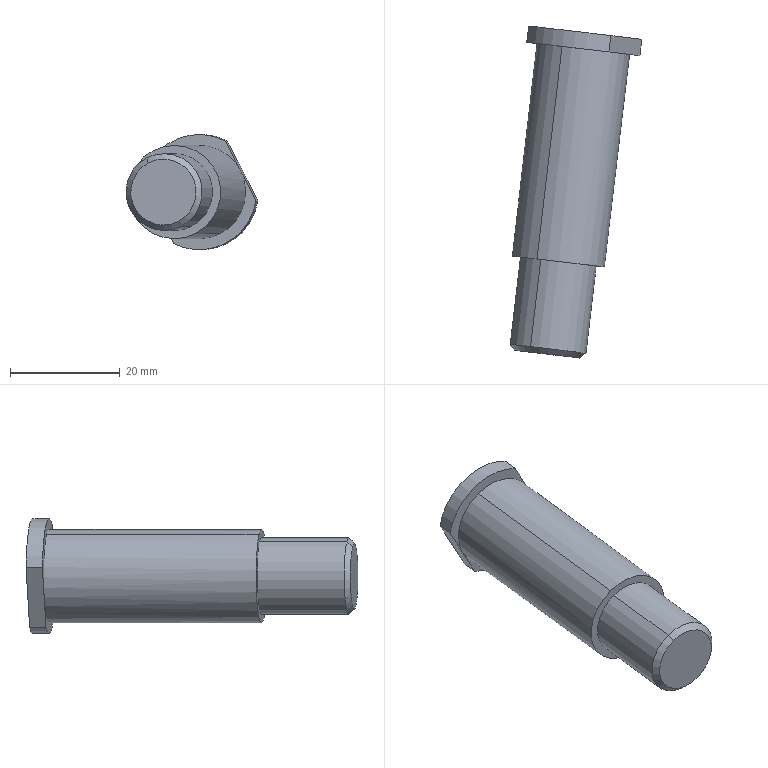Component | SolidWorks | 8TC-A17001-91-00UpperAndLowerPressAssembly-1_8TC-A17001-91-04PressureRollerAxis-1 | 1 solid | 16 faces | box 24.03 x 60.51 x 21 mm | volume 12387 mm3 | cylinder 7 | plane 7 | cone 2 | commonest cylinder face diameters 21 x3 14 x2 17 x2 | material Cr12MoV
build123d program:
from build123d import *

# Parameters (mm, degrees)
SKETCH1_R               = 10.5
BOSS_EXTRUDE1_DEPTH     = 3
SKETCH2_R               = 8.5
BOSS_EXTRUDE2_DEPTH     = 56
CUT_EXTRUDE1_DEPTH      = 61.84
CUT_EXTRUDE1_DEPTH_BACK = 61.84
SKETCH3_W               = 5
SKETCH3_H               = 5
SKETCH4_W               = 5
SKETCH4_H               = 17
CHAMFER1_SIZE           = 1


with BuildPart() as part:
    # Sketch1 → Boss-Extrude1 (new body)
    with BuildSketch(Plane(origin=(0, 0, 0), x_dir=(1, 0, 0), z_dir=(0, 1, 0))):
        with Locations(Location((0, 0, 0), (0, 0, 270))):
            Circle(SKETCH1_R)
    extrude(amount=BOSS_EXTRUDE1_DEPTH)

    # Sketch2 → Boss-Extrude2 (add)
    with BuildSketch(Plane(origin=(0, 3, 0), x_dir=(1, 0, 0), z_dir=(0, 1, 0))):
        with Locations(Location((0, 0, 0), (0, 0, 270))):
            Circle(SKETCH2_R)
    extrude(amount=BOSS_EXTRUDE2_DEPTH)

    # Sketch3 → Cut-Extrude1 (cut, two sides: drawn at the far end of the back side and taken through both)
    with BuildSketch(Plane.XY.offset(-CUT_EXTRUDE1_DEPTH_BACK)):
        with Locations((-11, 2.5)):
            Rectangle(SKETCH3_W, SKETCH3_H)
        with Locations((11, 2.5)):
            Rectangle(SKETCH3_W, SKETCH3_H)
    extrude(amount=CUT_EXTRUDE1_DEPTH + CUT_EXTRUDE1_DEPTH_BACK, mode=Mode.SUBTRACT)

    # Sketch4 → Cut-Revolve1 (revolve, cut)
    with BuildSketch(Plane.XY, mode=Mode.PRIVATE) as cut_revolve1_sk:
        with Locations((9.5, 50.5)):
            Rectangle(SKETCH4_W, SKETCH4_H)
    revolve(cut_revolve1_sk.sketch.rotate(Axis((0, 0, 0), (0, 1, 0)), 90), axis=Axis((0, 0, 0), (0, 1, 0)), mode=Mode.SUBTRACT)

    # Chamfer1
    chamfer1_edges = [part.edges().sort_by_distance(p)[0] for p in [
        (0, 59, 7),
    ]]
    chamfer(chamfer1_edges, length=CHAMFER1_SIZE)


solid = part.part

# Placed as in the assembly
solid = solid.moved(Location((3.937, -58.742, -52), (176.545, 27.162, 7.535)))
STEP:
#1=COLOUR_RGB('',0.7922,0.8196,0.9333);
#2=FILL_AREA_STYLE_COLOUR('',#1);
#3=FILL_AREA_STYLE('',(#2));
#4=SURFACE_STYLE_FILL_AREA(#3);
#5=SURFACE_SIDE_STYLE('',(#4));
#6=SURFACE_STYLE_USAGE(.BOTH.,#5);
#7=PRESENTATION_STYLE_ASSIGNMENT((#6));
#8=CARTESIAN_POINT('',(-0.2238,-4.607,-1.837));
#9=VERTEX_POINT('',#8);
#10=CARTESIAN_POINT('',(-0.008168,-4.632,-2.257));
#11=VERTEX_POINT('',#10);
#12=CARTESIAN_POINT('',(-0.116,-4.62,-2.047));
#13=DIRECTION('',(-0.1167,-0.9932,0.));
#14=DIRECTION('',(-0.4565,0.05363,0.8881));
#15=AXIS2_PLACEMENT_3D('',#12,#13,#14);
#16=CIRCLE('',#15,0.2362);
#17=EDGE_CURVE('',#9,#11,#16,.T.);
#18=ORIENTED_EDGE('',*,*,#17,.F.);
#19=CARTESIAN_POINT('',(-0.2372,-4.566,-1.802));
#20=VERTEX_POINT('',#19);
#21=CARTESIAN_POINT('',(-0.2372,-4.566,-1.802));
#22=DIRECTION('',(-0.2403,0.7402,0.628));
#23=VECTOR('',#22,39.37);
#24=LINE('',#21,#23);
#25=EDGE_CURVE('',#9,#20,#24,.T.);
#26=ORIENTED_EDGE('',*,*,#25,.T.);
#27=CARTESIAN_POINT('',(0.0144,-4.595,-2.292));
#28=VERTEX_POINT('',#27);
#29=CARTESIAN_POINT('',(-0.1114,-4.581,-2.047));
#30=DIRECTION('',(0.1167,0.9932,-0.));
#31=DIRECTION('',(-0.4565,0.05363,0.8881));
#32=AXIS2_PLACEMENT_3D('',#29,#30,#31);
#33=CIRCLE('',#32,0.2756);
#34=EDGE_CURVE('',#28,#20,#33,.T.);
#35=ORIENTED_EDGE('',*,*,#34,.F.);
#36=CARTESIAN_POINT('',(0.0144,-4.595,-2.292));
#37=DIRECTION('',(0.4053,0.6644,-0.628));
#38=VECTOR('',#37,39.37);
#39=LINE('',#36,#38);
#40=EDGE_CURVE('',#11,#28,#39,.T.);
#41=ORIENTED_EDGE('',*,*,#40,.F.);
#42=EDGE_LOOP('',(#18,#26,#35,#41));
#43=FACE_OUTER_BOUND('',#42,.T.);
#44=CARTESIAN_POINT('',(-0.1114,-4.581,-2.047));
#45=DIRECTION('',(0.1167,0.9932,-0.));
#46=DIRECTION('',(0.4565,-0.05363,-0.8881));
#47=AXIS2_PLACEMENT_3D('',#44,#45,#46);
#48=CONICAL_SURFACE('',#47,0.2756,0.7854);
#49=ADVANCED_FACE('',(#43),#48,.T.);
#50=ORIENTED_EDGE('',*,*,#34,.T.);
#51=CARTESIAN_POINT('',(-0.1637,-3.94,-1.802));
#52=VERTEX_POINT('',#51);
#53=CARTESIAN_POINT('',(0.02918,-2.298,-1.802));
#54=DIRECTION('',(0.1167,0.9932,-0.));
#55=VECTOR('',#54,39.37);
#56=LINE('',#53,#55);
#57=EDGE_CURVE('',#20,#52,#56,.T.);
#58=ORIENTED_EDGE('',*,*,#57,.T.);
#59=CARTESIAN_POINT('',(0.08789,-3.97,-2.292));
#60=VERTEX_POINT('',#59);
#61=CARTESIAN_POINT('',(-0.03792,-3.955,-2.047));
#62=DIRECTION('',(0.1167,0.9932,-0.));
#63=DIRECTION('',(0.4565,-0.05363,-0.8881));
#64=AXIS2_PLACEMENT_3D('',#61,#62,#63);
#65=CIRCLE('',#64,0.2756);
#66=EDGE_CURVE('',#60,#52,#65,.T.);
#67=ORIENTED_EDGE('',*,*,#66,.F.);
#68=CARTESIAN_POINT('',(0.2808,-2.327,-2.292));
#69=DIRECTION('',(0.1167,0.9932,-0.));
#70=VECTOR('',#69,39.37);
#71=LINE('',#68,#70);
#72=EDGE_CURVE('',#28,#60,#71,.T.);
#73=ORIENTED_EDGE('',*,*,#72,.F.);
#74=EDGE_LOOP('',(#50,#58,#67,#73));
#75=FACE_OUTER_BOUND('',#74,.T.);
#76=CARTESIAN_POINT('',(0.155,-2.313,-2.047));
#77=DIRECTION('',(0.1167,0.9932,-0.));
#78=DIRECTION('',(0.4565,-0.05363,-0.8881));
#79=AXIS2_PLACEMENT_3D('',#76,#77,#78);
#80=CYLINDRICAL_SURFACE('',#79,0.2756);
#81=ADVANCED_FACE('',(#75),#80,.T.);
#82=CARTESIAN_POINT('',(0.1148,-3.973,-2.344));
#83=VERTEX_POINT('',#82);
#84=CARTESIAN_POINT('',(-0.1907,-3.937,-1.75));
#85=VERTEX_POINT('',#84);
#86=CARTESIAN_POINT('',(-0.03792,-3.955,-2.047));
#87=DIRECTION('',(0.1167,0.9932,-0.));
#88=DIRECTION('',(0.4565,-0.05363,-0.8881));
#89=AXIS2_PLACEMENT_3D('',#86,#87,#88);
#90=CIRCLE('',#89,0.3346);
#91=EDGE_CURVE('',#83,#85,#90,.T.);
#92=ORIENTED_EDGE('',*,*,#91,.T.);
#93=CARTESIAN_POINT('',(-0.01156,-2.412,-1.75));
#94=VERTEX_POINT('',#93);
#95=CARTESIAN_POINT('',(-0.2688,-4.602,-1.75));
#96=DIRECTION('',(0.1167,0.9932,-0.));
#97=VECTOR('',#96,39.37);
#98=LINE('',#95,#97);
#99=EDGE_CURVE('',#85,#94,#98,.T.);
#100=ORIENTED_EDGE('',*,*,#99,.T.);
#101=CARTESIAN_POINT('',(-0.154,-2.395,-2.201));
#102=VERTEX_POINT('',#101);
#103=CARTESIAN_POINT('',(0.1412,-2.43,-2.047));
#104=DIRECTION('',(-0.1167,-0.9932,0.));
#105=DIRECTION('',(-0.4565,0.05363,0.8881));
#106=AXIS2_PLACEMENT_3D('',#103,#104,#105);
#107=CIRCLE('',#106,0.3346);
#108=EDGE_CURVE('',#94,#102,#107,.T.);
#109=ORIENTED_EDGE('',*,*,#108,.T.);
#110=CARTESIAN_POINT('',(0.294,-2.448,-2.344));
#111=VERTEX_POINT('',#110);
#112=CARTESIAN_POINT('',(0.1412,-2.43,-2.047));
#113=DIRECTION('',(-0.1167,-0.9932,0.));
#114=DIRECTION('',(-0.4565,0.05363,0.8881));
#115=AXIS2_PLACEMENT_3D('',#112,#113,#114);
#116=CIRCLE('',#115,0.3346);
#117=EDGE_CURVE('',#102,#111,#116,.T.);
#118=ORIENTED_EDGE('',*,*,#117,.T.);
#119=CARTESIAN_POINT('',(0.03676,-4.638,-2.344));
#120=DIRECTION('',(0.1167,0.9932,-0.));
#121=VECTOR('',#120,39.37);
#122=LINE('',#119,#121);
#123=EDGE_CURVE('',#83,#111,#122,.T.);
#124=ORIENTED_EDGE('',*,*,#123,.F.);
#125=EDGE_LOOP('',(#92,#100,#109,#118,#124));
#126=FACE_OUTER_BOUND('',#125,.T.);
#127=CARTESIAN_POINT('',(-0.116,-4.62,-2.047));
#128=DIRECTION('',(0.1167,0.9932,-0.));
#129=DIRECTION('',(0.4565,-0.05363,-0.8881));
#130=AXIS2_PLACEMENT_3D('',#127,#128,#129);
#131=CYLINDRICAL_SURFACE('',#130,0.3346);
#132=ADVANCED_FACE('',(#126),#131,.T.);
#133=CARTESIAN_POINT('',(0.3299,-2.452,-2.414));
#134=VERTEX_POINT('',#133);
#135=CARTESIAN_POINT('',(0.5472,-2.478,-2.109));
#136=VERTEX_POINT('',#135);
#137=CARTESIAN_POINT('',(0.1412,-2.43,-2.047));
#138=DIRECTION('',(-0.1167,-0.9932,0.));
#139=DIRECTION('',(-0.4565,0.05363,0.8881));
#140=AXIS2_PLACEMENT_3D('',#137,#138,#139);
#141=CIRCLE('',#140,0.4134);
#142=EDGE_CURVE('',#134,#136,#141,.T.);
#143=ORIENTED_EDGE('',*,*,#142,.F.);
#144=CARTESIAN_POINT('',(0.3437,-2.335,-2.414));
#145=VERTEX_POINT('',#144);
#146=CARTESIAN_POINT('',(0.3299,-2.452,-2.414));
#147=DIRECTION('',(0.1167,0.9932,-0.));
#148=VECTOR('',#147,39.37);
#149=LINE('',#146,#148);
#150=EDGE_CURVE('',#134,#145,#149,.T.);
#151=ORIENTED_EDGE('',*,*,#150,.T.);
#152=CARTESIAN_POINT('',(0.561,-2.36,-2.109));
#153=VERTEX_POINT('',#152);
#154=CARTESIAN_POINT('',(0.155,-2.313,-2.047));
#155=DIRECTION('',(-0.1167,-0.9932,0.));
#156=DIRECTION('',(-0.4565,0.05363,0.8881));
#157=AXIS2_PLACEMENT_3D('',#154,#155,#156);
#158=CIRCLE('',#157,0.4134);
#159=EDGE_CURVE('',#145,#153,#158,.T.);
#160=ORIENTED_EDGE('',*,*,#159,.T.);
#161=CARTESIAN_POINT('',(0.5472,-2.478,-2.109));
#162=DIRECTION('',(-0.1167,-0.9932,0.));
#163=VECTOR('',#162,39.37);
#164=LINE('',#161,#163);
#165=EDGE_CURVE('',#153,#136,#164,.T.);
#166=ORIENTED_EDGE('',*,*,#165,.T.);
#167=EDGE_LOOP('',(#143,#151,#160,#166));
#168=FACE_OUTER_BOUND('',#167,.T.);
#169=CARTESIAN_POINT('',(0.1412,-2.43,-2.047));
#170=DIRECTION('',(0.1167,0.9932,-0.));
#171=DIRECTION('',(0.4565,-0.05363,-0.8881));
#172=AXIS2_PLACEMENT_3D('',#169,#170,#171);
#173=CYLINDRICAL_SURFACE('',#172,0.4134);
#174=ADVANCED_FACE('',(#168),#173,.T.);
#175=ORIENTED_EDGE('',*,*,#150,.F.);
#176=CARTESIAN_POINT('',(-0.04317,-2.408,-2.417));
#177=VERTEX_POINT('',#176);
#178=CARTESIAN_POINT('',(0.1412,-2.43,-2.047));
#179=DIRECTION('',(-0.1167,-0.9932,0.));
#180=DIRECTION('',(-0.4565,0.05363,0.8881));
#181=AXIS2_PLACEMENT_3D('',#178,#179,#180);
#182=CIRCLE('',#181,0.4134);
#183=EDGE_CURVE('',#177,#134,#182,.T.);
#184=ORIENTED_EDGE('',*,*,#183,.F.);
#185=CARTESIAN_POINT('',(-0.02939,-2.291,-2.417));
#186=VERTEX_POINT('',#185);
#187=CARTESIAN_POINT('',(-0.04317,-2.408,-2.417));
#188=DIRECTION('',(0.1167,0.9932,-0.));
#189=VECTOR('',#188,39.37);
#190=LINE('',#187,#189);
#191=EDGE_CURVE('',#177,#186,#190,.T.);
#192=ORIENTED_EDGE('',*,*,#191,.T.);
#193=CARTESIAN_POINT('',(0.155,-2.313,-2.047));
#194=DIRECTION('',(-0.1167,-0.9932,0.));
#195=DIRECTION('',(-0.4565,0.05363,0.8881));
#196=AXIS2_PLACEMENT_3D('',#193,#194,#195);
#197=CIRCLE('',#196,0.4134);
#198=EDGE_CURVE('',#186,#145,#197,.T.);
#199=ORIENTED_EDGE('',*,*,#198,.T.);
#200=EDGE_LOOP('',(#175,#184,#192,#199));
#201=FACE_OUTER_BOUND('',#200,.T.);
#202=CARTESIAN_POINT('',(0.1412,-2.43,-2.047));
#203=DIRECTION('',(0.1167,0.9932,-0.));
#204=DIRECTION('',(0.4565,-0.05363,-0.8881));
#205=AXIS2_PLACEMENT_3D('',#202,#203,#204);
#206=CYLINDRICAL_SURFACE('',#205,0.4134);
#207=ADVANCED_FACE('',(#201),#206,.T.);
#208=CARTESIAN_POINT('',(-0.154,-2.395,-2.201));
#209=DIRECTION('',(-0.4565,0.05363,0.8881));
#210=VECTOR('',#209,39.37);
#211=LINE('',#208,#210);
#212=EDGE_CURVE('',#177,#102,#211,.T.);
#213=ORIENTED_EDGE('',*,*,#212,.F.);
#214=ORIENTED_EDGE('',*,*,#183,.T.);
#215=ORIENTED_EDGE('',*,*,#142,.T.);
#216=CARTESIAN_POINT('',(0.4364,-2.465,-1.893));
#217=VERTEX_POINT('',#216);
#218=CARTESIAN_POINT('',(0.4364,-2.465,-1.893));
#219=DIRECTION('',(0.4565,-0.05363,-0.8881));
#220=VECTOR('',#219,39.37);
#221=LINE('',#218,#220);
#222=EDGE_CURVE('',#217,#136,#221,.T.);
#223=ORIENTED_EDGE('',*,*,#222,.F.);
#224=CARTESIAN_POINT('',(0.1412,-2.43,-2.047));
#225=DIRECTION('',(-0.1167,-0.9932,0.));
#226=DIRECTION('',(-0.4565,0.05363,0.8881));
#227=AXIS2_PLACEMENT_3D('',#224,#225,#226);
#228=CIRCLE('',#227,0.3346);
#229=EDGE_CURVE('',#111,#217,#228,.T.);
#230=ORIENTED_EDGE('',*,*,#229,.F.);
#231=ORIENTED_EDGE('',*,*,#117,.F.);
#232=EDGE_LOOP('',(#213,#214,#215,#223,#230,#231));
#233=FACE_OUTER_BOUND('',#232,.T.);
#234=CARTESIAN_POINT('',(0.1412,-2.43,-2.047));
#235=DIRECTION('',(-0.1167,-0.9932,-0.));
#236=DIRECTION('',(-0.4565,0.05363,0.8881));
#237=AXIS2_PLACEMENT_3D('',#234,#235,#236);
#238=PLANE('',#237);
#239=ADVANCED_FACE('',(#233),#238,.T.);
#240=CARTESIAN_POINT('',(0.3394,-2.334,-1.678));
#241=VERTEX_POINT('',#240);
#242=CARTESIAN_POINT('',(-0.251,-2.265,-1.986));
#243=VERTEX_POINT('',#242);
#244=CARTESIAN_POINT('',(0.155,-2.313,-2.047));
#245=DIRECTION('',(-0.1167,-0.9932,0.));
#246=DIRECTION('',(-0.4565,0.05363,0.8881));
#247=AXIS2_PLACEMENT_3D('',#244,#245,#246);
#248=CIRCLE('',#247,0.4134);
#249=EDGE_CURVE('',#241,#243,#248,.T.);
#250=ORIENTED_EDGE('',*,*,#249,.T.);
#251=CARTESIAN_POINT('',(-0.2647,-2.382,-1.986));
#252=VERTEX_POINT('',#251);
#253=CARTESIAN_POINT('',(-0.2647,-2.382,-1.986));
#254=DIRECTION('',(-0.1167,-0.9932,0.));
#255=VECTOR('',#254,39.37);
#256=LINE('',#253,#255);
#257=EDGE_CURVE('',#243,#252,#256,.T.);
#258=ORIENTED_EDGE('',*,*,#257,.T.);
#259=CARTESIAN_POINT('',(0.3256,-2.452,-1.678));
#260=VERTEX_POINT('',#259);
#261=CARTESIAN_POINT('',(0.1412,-2.43,-2.047));
#262=DIRECTION('',(-0.1167,-0.9932,0.));
#263=DIRECTION('',(-0.4565,0.05363,0.8881));
#264=AXIS2_PLACEMENT_3D('',#261,#262,#263);
#265=CIRCLE('',#264,0.4134);
#266=EDGE_CURVE('',#260,#252,#265,.T.);
#267=ORIENTED_EDGE('',*,*,#266,.F.);
#268=CARTESIAN_POINT('',(0.3256,-2.452,-1.678));
#269=DIRECTION('',(0.1167,0.9932,-0.));
#270=VECTOR('',#269,39.37);
#271=LINE('',#268,#270);
#272=EDGE_CURVE('',#260,#241,#271,.T.);
#273=ORIENTED_EDGE('',*,*,#272,.T.);
#274=EDGE_LOOP('',(#250,#258,#267,#273));
#275=FACE_OUTER_BOUND('',#274,.T.);
#276=CARTESIAN_POINT('',(0.1412,-2.43,-2.047));
#277=DIRECTION('',(0.1167,0.9932,-0.));
#278=DIRECTION('',(0.4565,-0.05363,-0.8881));
#279=AXIS2_PLACEMENT_3D('',#276,#277,#278);
#280=CYLINDRICAL_SURFACE('',#279,0.4134);
#281=ADVANCED_FACE('',(#275),#280,.T.);
#282=CARTESIAN_POINT('',(-0.154,-2.395,-2.201));
#283=DIRECTION('',(-0.4565,0.05363,0.8881));
#284=VECTOR('',#283,39.37);
#285=LINE('',#282,#284);
#286=EDGE_CURVE('',#102,#252,#285,.T.);
#287=ORIENTED_EDGE('',*,*,#286,.F.);
#288=ORIENTED_EDGE('',*,*,#108,.F.);
#289=CARTESIAN_POINT('',(0.1412,-2.43,-2.047));
#290=DIRECTION('',(-0.1167,-0.9932,0.));
#291=DIRECTION('',(-0.4565,0.05363,0.8881));
#292=AXIS2_PLACEMENT_3D('',#289,#290,#291);
#293=CIRCLE('',#292,0.3346);
#294=EDGE_CURVE('',#217,#94,#293,.T.);
#295=ORIENTED_EDGE('',*,*,#294,.F.);
#296=CARTESIAN_POINT('',(0.4364,-2.465,-1.893));
#297=DIRECTION('',(0.4565,-0.05363,-0.8881));
#298=VECTOR('',#297,39.37);
#299=LINE('',#296,#298);
#300=EDGE_CURVE('',#260,#217,#299,.T.);
#301=ORIENTED_EDGE('',*,*,#300,.F.);
#302=ORIENTED_EDGE('',*,*,#266,.T.);
#303=EDGE_LOOP('',(#287,#288,#295,#301,#302));
#304=FACE_OUTER_BOUND('',#303,.T.);
#305=CARTESIAN_POINT('',(0.1412,-2.43,-2.047));
#306=DIRECTION('',(-0.1167,-0.9932,-0.));
#307=DIRECTION('',(-0.4565,0.05363,0.8881));
#308=AXIS2_PLACEMENT_3D('',#305,#306,#307);
#309=PLANE('',#308);
#310=ADVANCED_FACE('',(#304),#309,.T.);
#311=ORIENTED_EDGE('',*,*,#198,.F.);
#312=CARTESIAN_POINT('',(0.04854,-2.3,-2.568));
#313=DIRECTION('',(-0.4565,0.05363,0.8881));
#314=VECTOR('',#313,39.37);
#315=LINE('',#312,#314);
#316=EDGE_CURVE('',#186,#243,#315,.T.);
#317=ORIENTED_EDGE('',*,*,#316,.T.);
#318=ORIENTED_EDGE('',*,*,#249,.F.);
#319=CARTESIAN_POINT('',(0.6389,-2.37,-2.261));
#320=DIRECTION('',(-0.4565,0.05363,0.8881));
#321=VECTOR('',#320,39.37);
#322=LINE('',#319,#321);
#323=EDGE_CURVE('',#153,#241,#322,.T.);
#324=ORIENTED_EDGE('',*,*,#323,.F.);
#325=ORIENTED_EDGE('',*,*,#159,.F.);
#326=EDGE_LOOP('',(#311,#317,#318,#324,#325));
#327=FACE_OUTER_BOUND('',#326,.T.);
#328=CARTESIAN_POINT('',(0.155,-2.313,-2.047));
#329=DIRECTION('',(-0.1167,-0.9932,-0.));
#330=DIRECTION('',(-0.4565,0.05363,0.8881));
#331=AXIS2_PLACEMENT_3D('',#328,#329,#330);
#332=PLANE('',#331);
#333=ADVANCED_FACE('',(#327),#332,.F.);
#334=ORIENTED_EDGE('',*,*,#99,.F.);
#335=CARTESIAN_POINT('',(-0.03792,-3.955,-2.047));
#336=DIRECTION('',(0.1167,0.9932,-0.));
#337=DIRECTION('',(0.4565,-0.05363,-0.8881));
#338=AXIS2_PLACEMENT_3D('',#335,#336,#337);
#339=CIRCLE('',#338,0.3346);
#340=EDGE_CURVE('',#85,#83,#339,.T.);
#341=ORIENTED_EDGE('',*,*,#340,.T.);
#342=ORIENTED_EDGE('',*,*,#123,.T.);
#343=ORIENTED_EDGE('',*,*,#229,.T.);
#344=ORIENTED_EDGE('',*,*,#294,.T.);
#345=EDGE_LOOP('',(#334,#341,#342,#343,#344));
#346=FACE_OUTER_BOUND('',#345,.T.);
#347=CARTESIAN_POINT('',(-0.116,-4.62,-2.047));
#348=DIRECTION('',(0.1167,0.9932,-0.));
#349=DIRECTION('',(0.4565,-0.05363,-0.8881));
#350=AXIS2_PLACEMENT_3D('',#347,#348,#349);
#351=CYLINDRICAL_SURFACE('',#350,0.3346);
#352=ADVANCED_FACE('',(#346),#351,.T.);
#353=ORIENTED_EDGE('',*,*,#300,.T.);
#354=ORIENTED_EDGE('',*,*,#222,.T.);
#355=ORIENTED_EDGE('',*,*,#165,.F.);
#356=ORIENTED_EDGE('',*,*,#323,.T.);
#357=ORIENTED_EDGE('',*,*,#272,.F.);
#358=EDGE_LOOP('',(#353,#354,#355,#356,#357));
#359=FACE_OUTER_BOUND('',#358,.T.);
#360=CARTESIAN_POINT('',(0.6159,-2.565,-2.261));
#361=DIRECTION('',(-0.882,0.1036,-0.4596));
#362=DIRECTION('',(0.4565,-0.05363,-0.8881));
#363=AXIS2_PLACEMENT_3D('',#360,#361,#362);
#364=PLANE('',#363);
#365=ADVANCED_FACE('',(#359),#364,.F.);
#366=ORIENTED_EDGE('',*,*,#212,.T.);
#367=ORIENTED_EDGE('',*,*,#286,.T.);
#368=ORIENTED_EDGE('',*,*,#257,.F.);
#369=ORIENTED_EDGE('',*,*,#316,.F.);
#370=ORIENTED_EDGE('',*,*,#191,.F.);
#371=EDGE_LOOP('',(#366,#367,#368,#369,#370));
#372=FACE_OUTER_BOUND('',#371,.T.);
#373=CARTESIAN_POINT('',(0.02557,-2.496,-2.568));
#374=DIRECTION('',(0.882,-0.1036,0.4596));
#375=DIRECTION('',(-0.4565,0.05363,0.8881));
#376=AXIS2_PLACEMENT_3D('',#373,#374,#375);
#377=PLANE('',#376);
#378=ADVANCED_FACE('',(#372),#377,.F.);
#379=ORIENTED_EDGE('',*,*,#66,.T.);
#380=CARTESIAN_POINT('',(-0.03792,-3.955,-2.047));
#381=DIRECTION('',(0.1167,0.9932,-0.));
#382=DIRECTION('',(0.4565,-0.05363,-0.8881));
#383=AXIS2_PLACEMENT_3D('',#380,#381,#382);
#384=CIRCLE('',#383,0.2756);
#385=EDGE_CURVE('',#52,#60,#384,.T.);
#386=ORIENTED_EDGE('',*,*,#385,.T.);
#387=EDGE_LOOP('',(#379,#386));
#388=FACE_BOUND('',#387,.T.);
#389=ORIENTED_EDGE('',*,*,#91,.F.);
#390=ORIENTED_EDGE('',*,*,#340,.F.);
#391=EDGE_LOOP('',(#389,#390));
#392=FACE_OUTER_BOUND('',#391,.T.);
#393=CARTESIAN_POINT('',(-0.281,-3.926,-2.174));
#394=DIRECTION('',(0.1167,0.9932,0.));
#395=DIRECTION('',(0.4565,-0.05363,-0.8881));
#396=AXIS2_PLACEMENT_3D('',#393,#394,#395);
#397=PLANE('',#396);
#398=ADVANCED_FACE('',(#388,#392),#397,.F.);
#399=ORIENTED_EDGE('',*,*,#57,.F.);
#400=CARTESIAN_POINT('',(-0.1114,-4.581,-2.047));
#401=DIRECTION('',(0.1167,0.9932,-0.));
#402=DIRECTION('',(-0.4565,0.05363,0.8881));
#403=AXIS2_PLACEMENT_3D('',#400,#401,#402);
#404=CIRCLE('',#403,0.2756);
#405=EDGE_CURVE('',#20,#28,#404,.T.);
#406=ORIENTED_EDGE('',*,*,#405,.T.);
#407=ORIENTED_EDGE('',*,*,#72,.T.);
#408=ORIENTED_EDGE('',*,*,#385,.F.);
#409=EDGE_LOOP('',(#399,#406,#407,#408));
#410=FACE_OUTER_BOUND('',#409,.T.);
#411=CARTESIAN_POINT('',(0.155,-2.313,-2.047));
#412=DIRECTION('',(0.1167,0.9932,-0.));
#413=DIRECTION('',(0.4565,-0.05363,-0.8881));
#414=AXIS2_PLACEMENT_3D('',#411,#412,#413);
#415=CYLINDRICAL_SURFACE('',#414,0.2756);
#416=ADVANCED_FACE('',(#410),#415,.T.);
#417=CARTESIAN_POINT('',(-0.116,-4.62,-2.047));
#418=DIRECTION('',(-0.1167,-0.9932,0.));
#419=DIRECTION('',(-0.4565,0.05363,0.8881));
#420=AXIS2_PLACEMENT_3D('',#417,#418,#419);
#421=CIRCLE('',#420,0.2362);
#422=EDGE_CURVE('',#11,#9,#421,.T.);
#423=ORIENTED_EDGE('',*,*,#422,.T.);
#424=ORIENTED_EDGE('',*,*,#17,.T.);
#425=EDGE_LOOP('',(#423,#424));
#426=FACE_OUTER_BOUND('',#425,.T.);
#427=CARTESIAN_POINT('',(-0.116,-4.62,-2.047));
#428=DIRECTION('',(-0.1167,-0.9932,-0.));
#429=DIRECTION('',(-0.4565,0.05363,0.8881));
#430=AXIS2_PLACEMENT_3D('',#427,#428,#429);
#431=PLANE('',#430);
#432=ADVANCED_FACE('',(#426),#431,.T.);
#433=ORIENTED_EDGE('',*,*,#25,.F.);
#434=ORIENTED_EDGE('',*,*,#422,.F.);
#435=ORIENTED_EDGE('',*,*,#40,.T.);
#436=ORIENTED_EDGE('',*,*,#405,.F.);
#437=EDGE_LOOP('',(#433,#434,#435,#436));
#438=FACE_OUTER_BOUND('',#437,.T.);
#439=CARTESIAN_POINT('',(-0.1114,-4.581,-2.047));
#440=DIRECTION('',(0.1167,0.9932,-0.));
#441=DIRECTION('',(0.4565,-0.05363,-0.8881));
#442=AXIS2_PLACEMENT_3D('',#439,#440,#441);
#443=CONICAL_SURFACE('',#442,0.2756,0.7854);
#444=ADVANCED_FACE('',(#438),#443,.T.);
#445=CLOSED_SHELL('',(#49,#81,#132,#174,#207,#239,#281,#310,#333,#352,#365,#378,#398,#416,#432,#444));
#446=MANIFOLD_SOLID_BREP('',#445);
#447=STYLED_ITEM('',(#7),#446);
#448=(LENGTH_UNIT()NAMED_UNIT(*)SI_UNIT($,.METRE.));
#449=LENGTH_MEASURE_WITH_UNIT(LENGTH_MEASURE(0.0254),#448);
#450=DIMENSIONAL_EXPONENTS(1.,0.,0.,0.,0.,0.,0.);
#451=(CONVERSION_BASED_UNIT('',#449)LENGTH_UNIT()NAMED_UNIT(#450));
#452=UNCERTAINTY_MEASURE_WITH_UNIT(LENGTH_MEASURE(0.00001),#451,'','');
#453=(NAMED_UNIT(*)PLANE_ANGLE_UNIT()SI_UNIT($,.RADIAN.));
#454=(NAMED_UNIT(*)SI_UNIT($,.STERADIAN.)SOLID_ANGLE_UNIT());
#455=(GEOMETRIC_REPRESENTATION_CONTEXT(3)GLOBAL_UNCERTAINTY_ASSIGNED_CONTEXT((#452))GLOBAL_UNIT_ASSIGNED_CONTEXT((#451,#453,#454))REPRESENTATION_CONTEXT('',''));
#456=MECHANICAL_DESIGN_GEOMETRIC_PRESENTATION_REPRESENTATION('',(#447),#455);
#457=CARTESIAN_POINT('',(0.,0.,0.));
#458=DIRECTION('',(0.,0.,1.));
#459=DIRECTION('',(1.,0.,0.));
#460=AXIS2_PLACEMENT_3D('',#457,#458,#459);
#461=(LENGTH_UNIT()NAMED_UNIT(*)SI_UNIT($,.METRE.));
#462=LENGTH_MEASURE_WITH_UNIT(LENGTH_MEASURE(0.0254),#461);
#463=DIMENSIONAL_EXPONENTS(1.,0.,0.,0.,0.,0.,0.);
#464=(CONVERSION_BASED_UNIT('',#462)LENGTH_UNIT()NAMED_UNIT(#463));
#465=UNCERTAINTY_MEASURE_WITH_UNIT(LENGTH_MEASURE(0.00001),#464,'','');
#466=(NAMED_UNIT(*)PLANE_ANGLE_UNIT()SI_UNIT($,.RADIAN.));
#467=(NAMED_UNIT(*)SI_UNIT($,.STERADIAN.)SOLID_ANGLE_UNIT());
#468=(GEOMETRIC_REPRESENTATION_CONTEXT(3)GLOBAL_UNCERTAINTY_ASSIGNED_CONTEXT((#465))GLOBAL_UNIT_ASSIGNED_CONTEXT((#464,#466,#467))REPRESENTATION_CONTEXT('',''));
#469=ADVANCED_BREP_SHAPE_REPRESENTATION('',(#446,#460),#468);
#470=PRESENTATION_LAYER_ASSIGNMENT('','',(#447));